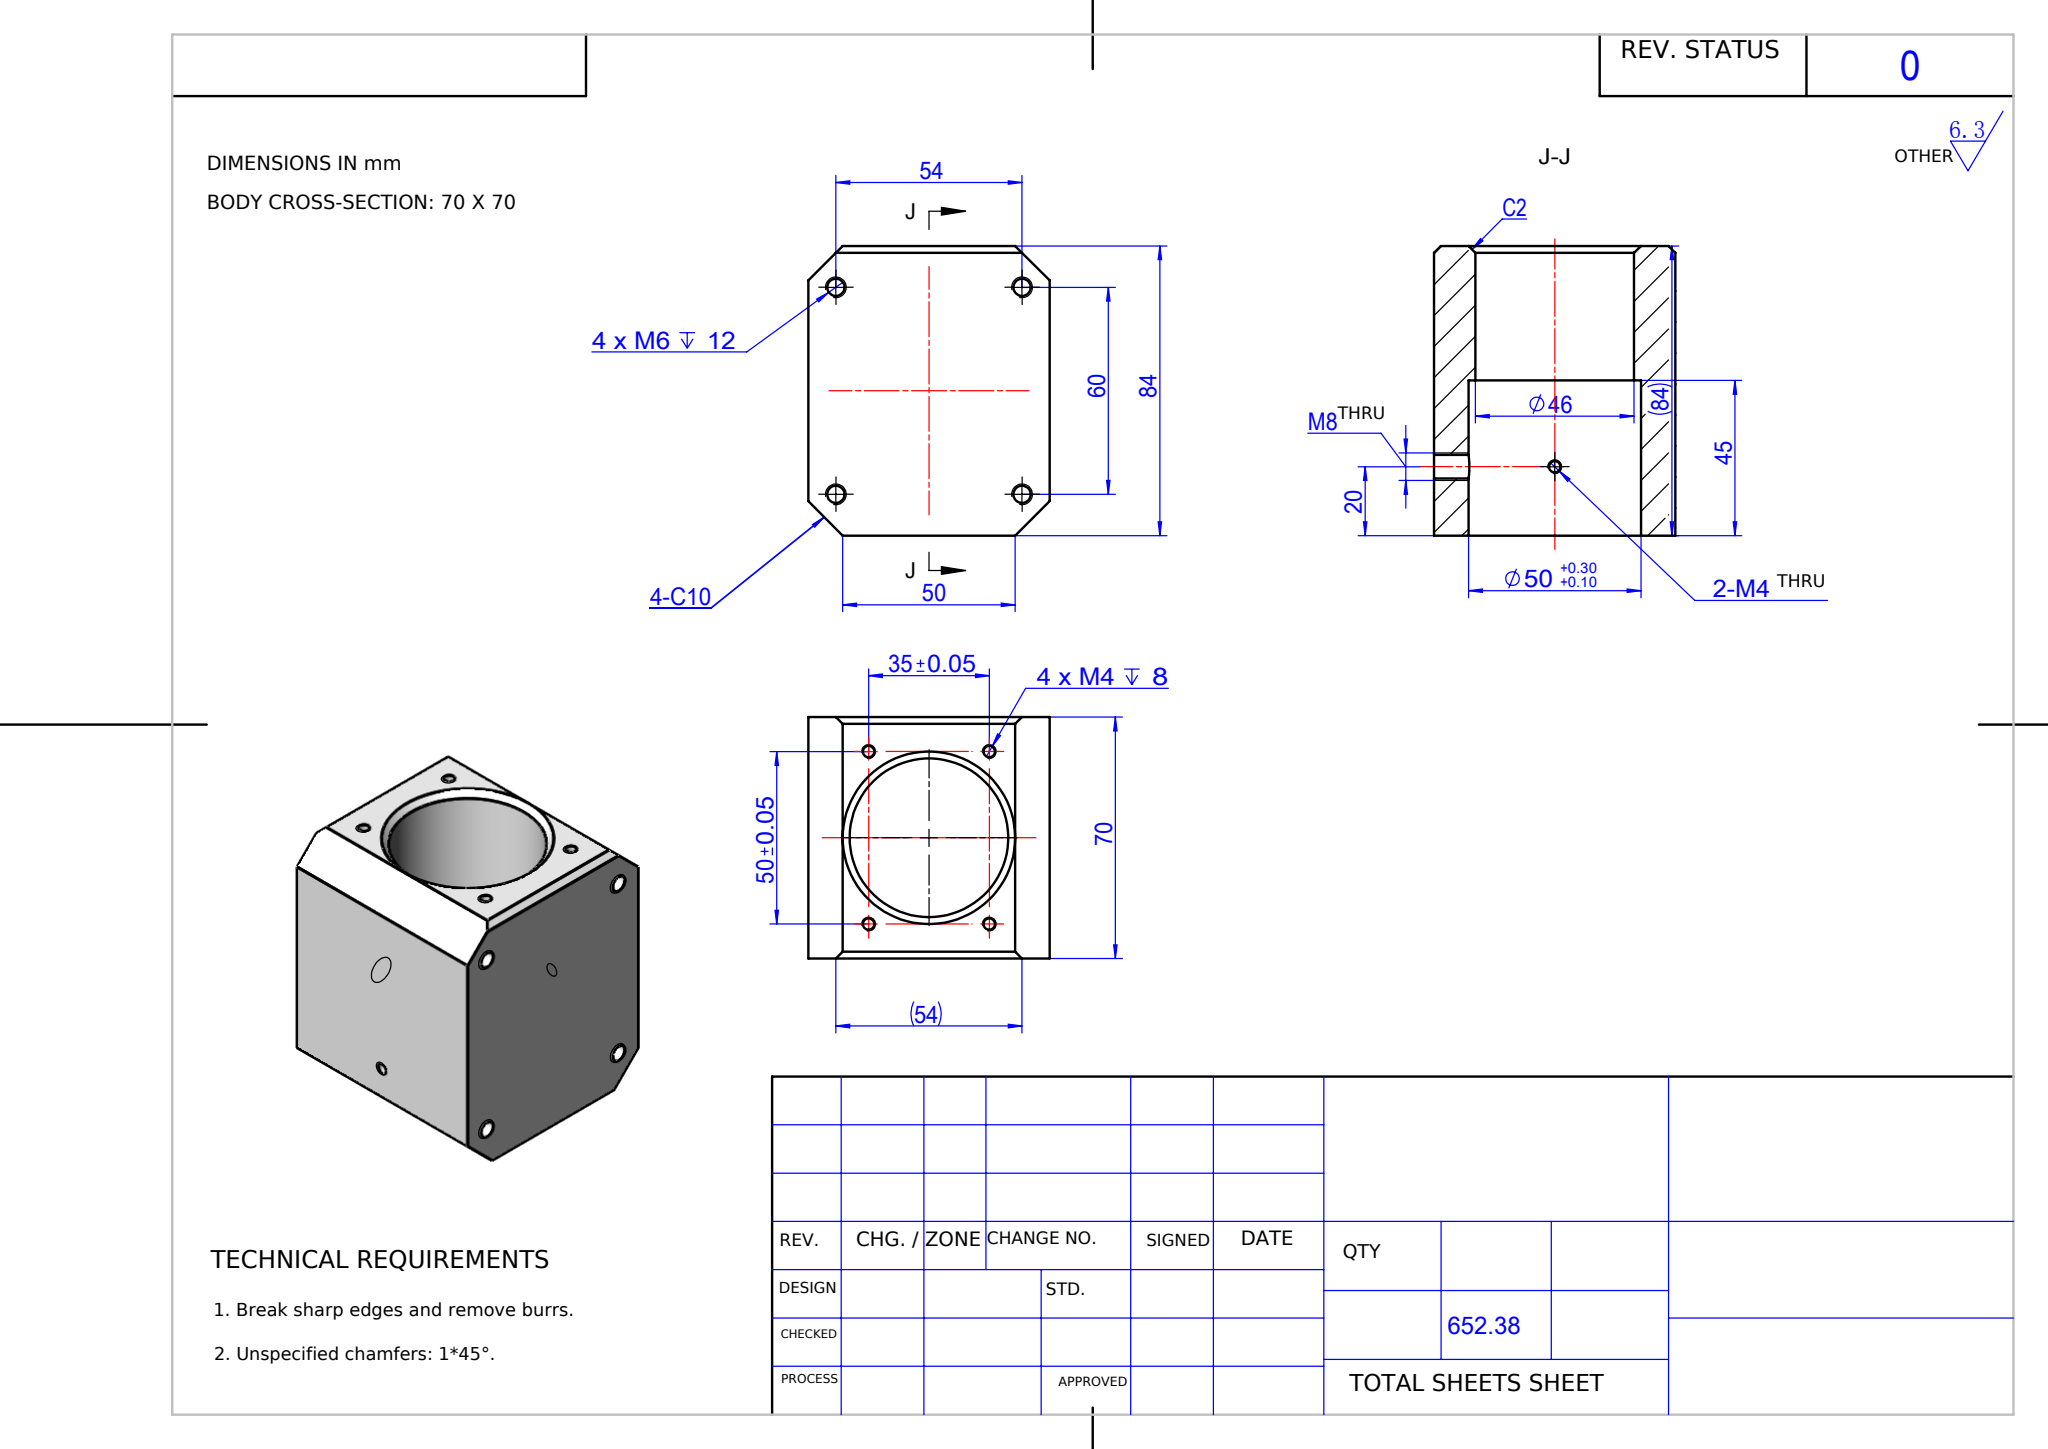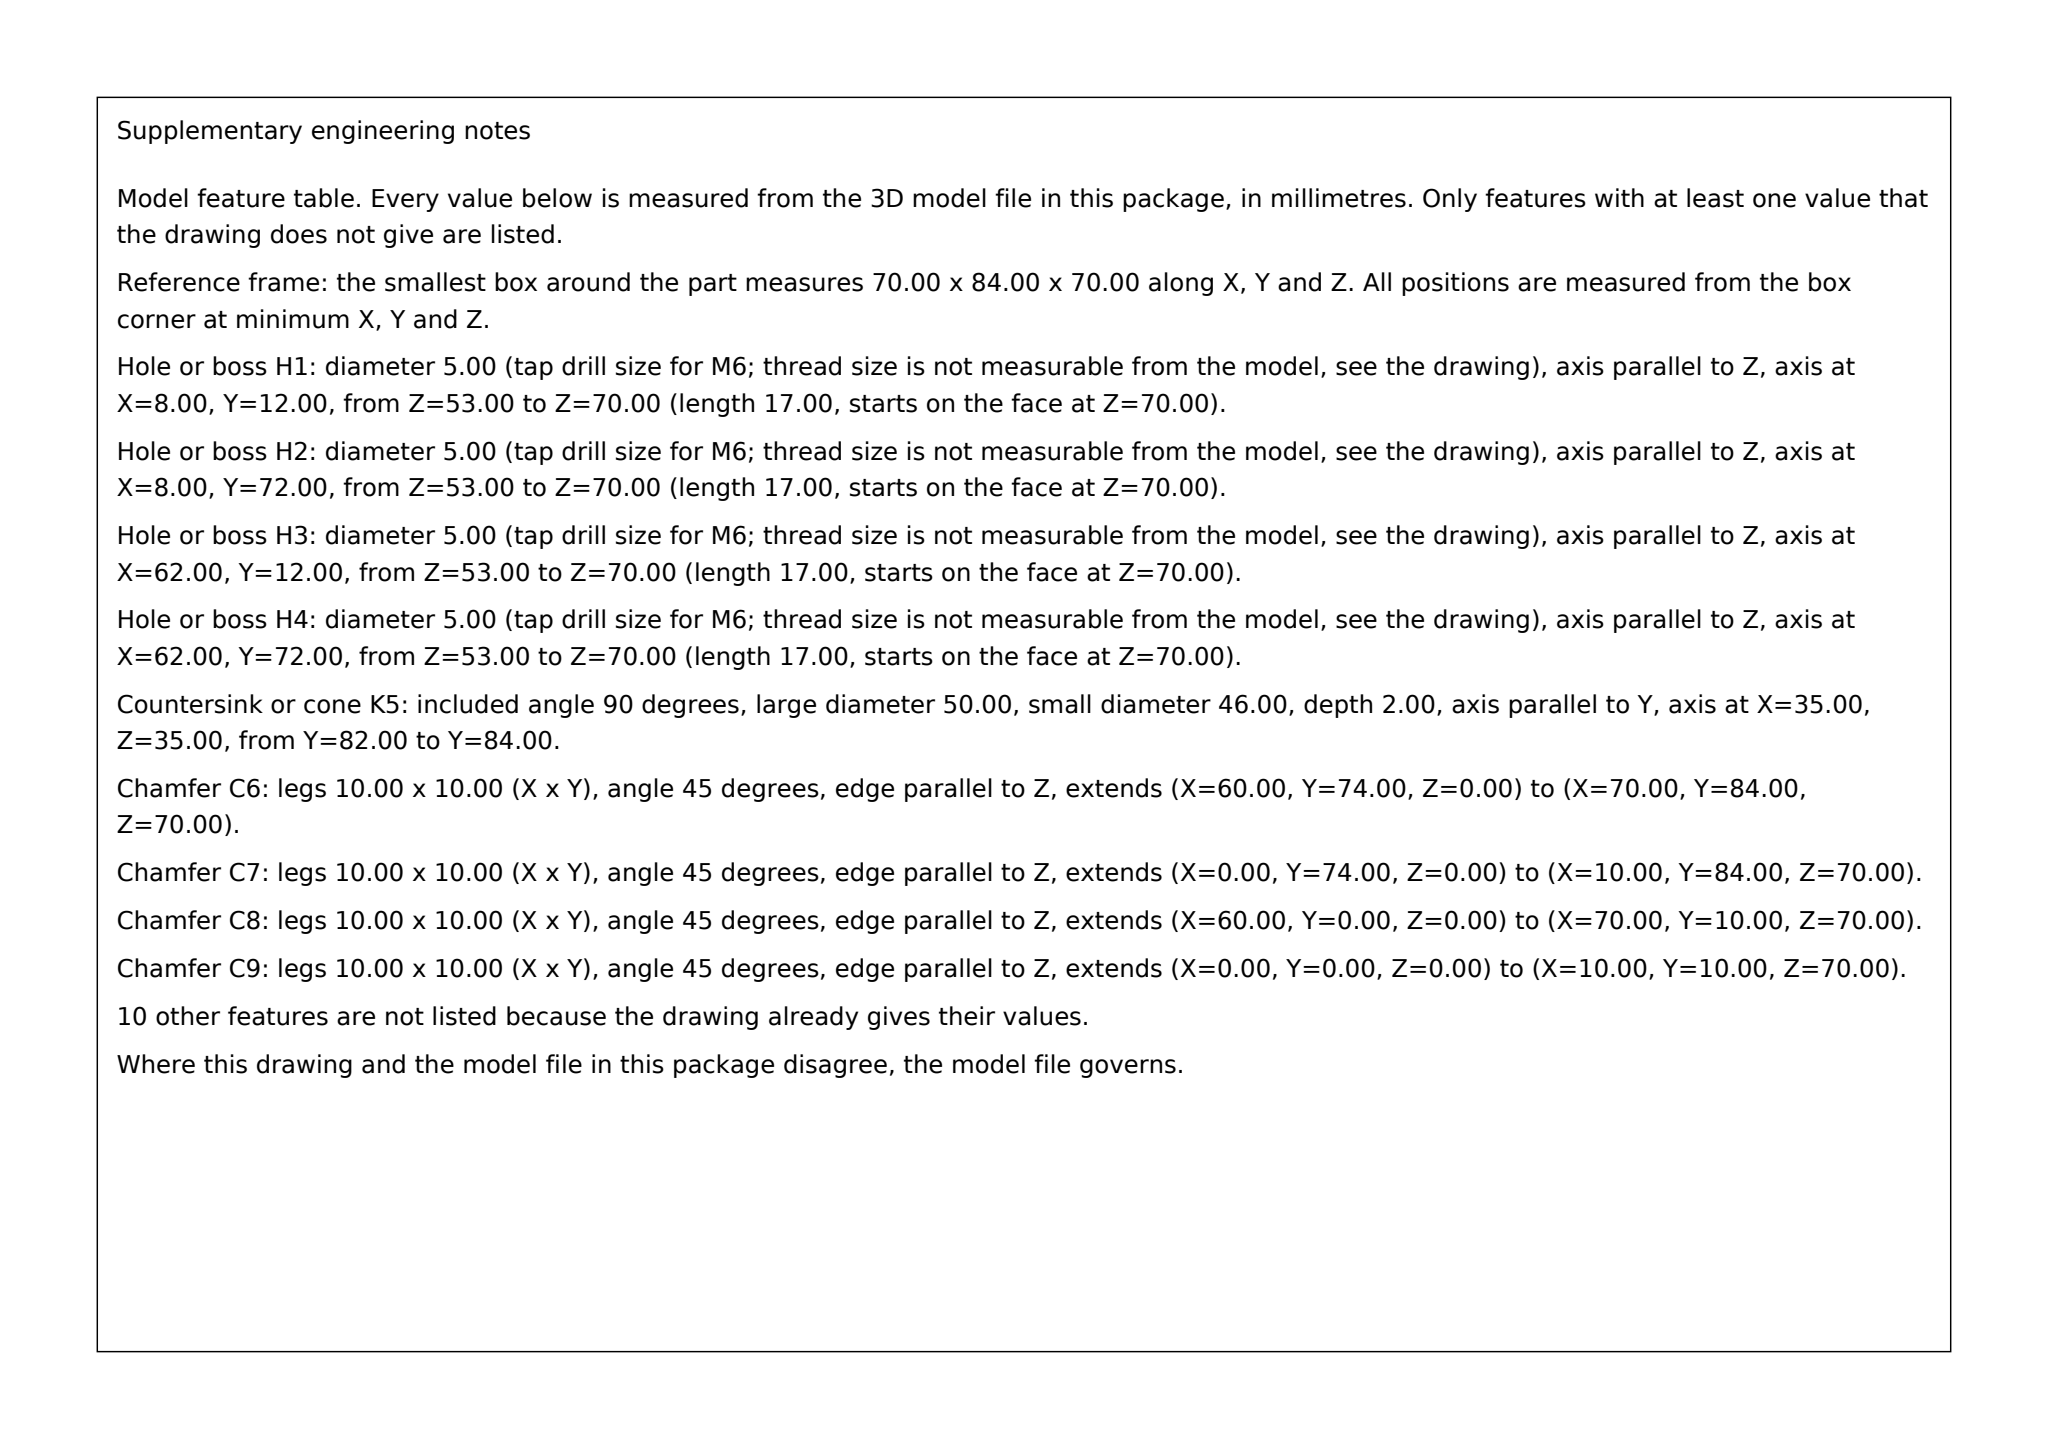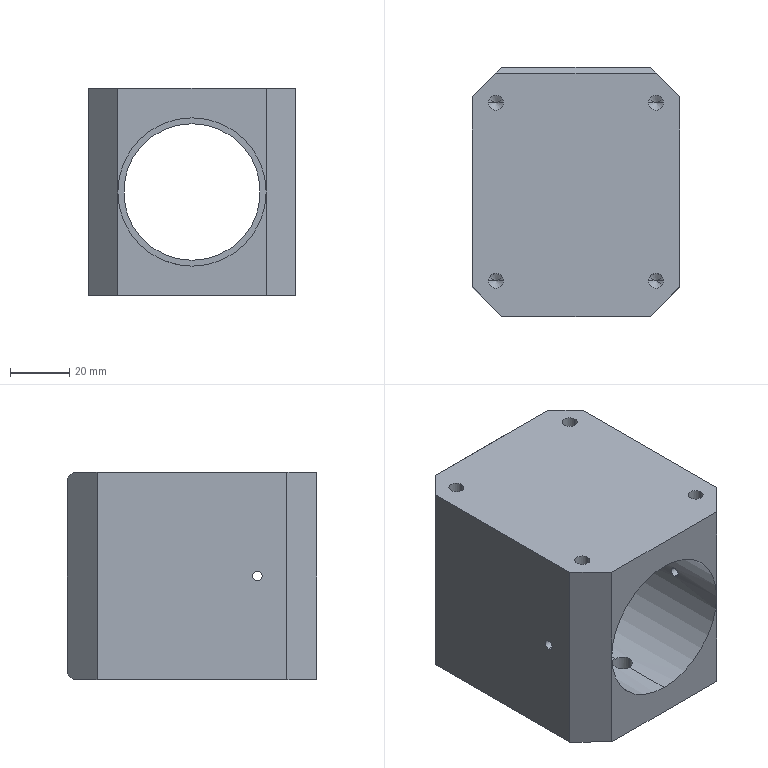Part | SolidWorks | mm | 1 solid | 55 faces | box 70 x 84 x 70 mm | volume 241621 mm3 | cylinder 26 | plane 19 | cone 10 | commonest cylinder face diameters 3.3 x12 5 x8 6.8 x2 46 x2 50 x2